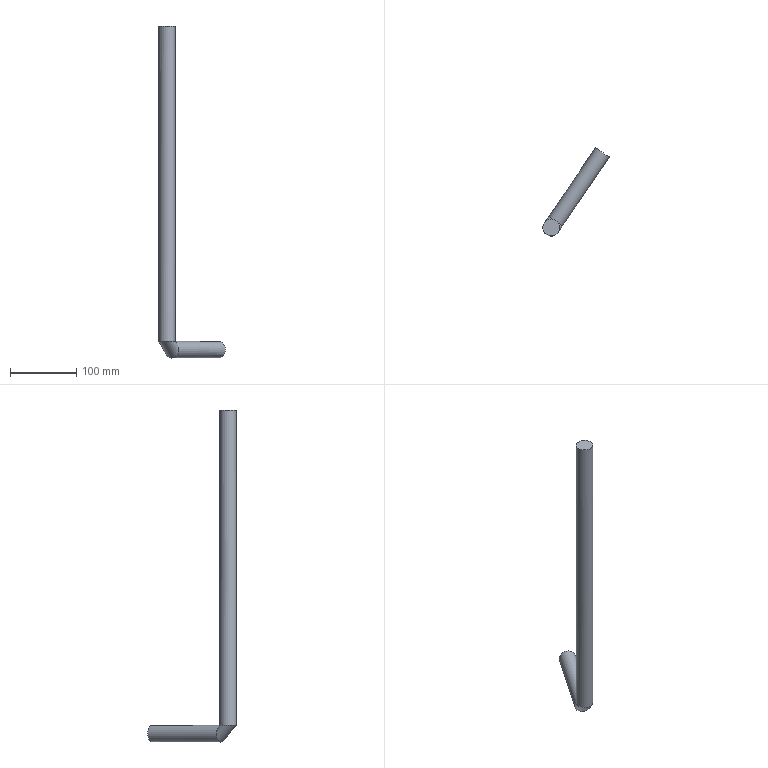Component | NX | PIN | 1 solid | 5 faces | box 100.07 x 133.28 x 500 mm | volume 304163 mm3 | cylinder 2 | plane 2 | torus 1 | commonest cylinder face diameters 25 x2
STEP:
#1=CARTESIAN_POINT('',(0.,0.,0.));
#2=DIRECTION('',(0.,0.,1.));
#3=DIRECTION('',(1.,0.,0.));
#4=AXIS2_PLACEMENT_3D('',#1,#2,#3);
#5=CARTESIAN_POINT('',(-196.929,1175.934,-262.682));
#6=VERTEX_POINT('',#5);
#7=CARTESIAN_POINT('',(-186.587,1168.913,-262.682));
#8=DIRECTION('',(0.5617,0.8274,-0.));
#9=DIRECTION('',(-0.8274,0.5617,0.));
#10=AXIS2_PLACEMENT_3D('',#7,#8,#9);
#11=CIRCLE('',#10,12.5);
#12=CARTESIAN_POINT('',(-256.797,1065.494,-262.682));
#13=DIRECTION('',(0.5617,0.8274,0.));
#14=DIRECTION('',(-0.8274,0.5617,0.));
#15=AXIS2_PLACEMENT_3D('',#12,#13,#14);
#16=CYLINDRICAL_SURFACE('',#15,12.5);
#17=CARTESIAN_POINT('',(0.,125.));
#18=DIRECTION('',(1.,0.));
#19=VECTOR('',#18,1.);
#20=LINE('',#17,#19);
#21=(GEOMETRIC_REPRESENTATION_CONTEXT(2)PARAMETRIC_REPRESENTATION_CONTEXT()REPRESENTATION_CONTEXT('',''));
#22=DEFINITIONAL_REPRESENTATION('',(#20),#21);
#23=PCURVE('',#16,#22);
#24=CARTESIAN_POINT('',(-186.587,1168.913,-262.682));
#25=DIRECTION('',(0.5617,0.8274,-0.));
#26=DIRECTION('',(-0.,-0.,-1.));
#27=AXIS2_PLACEMENT_3D('',#24,#25,#26);
#28=PLANE('',#27);
#29=CARTESIAN_POINT('',(0.,0.));
#30=DIRECTION('',(0.,1.));
#31=AXIS2_PLACEMENT_2D('',#29,#30);
#32=CIRCLE('',#31,12.5);
#33=(GEOMETRIC_REPRESENTATION_CONTEXT(2)PARAMETRIC_REPRESENTATION_CONTEXT()REPRESENTATION_CONTEXT('',''));
#34=DEFINITIONAL_REPRESENTATION('',(#32),#33);
#35=PCURVE('',#28,#34);
#36=SURFACE_CURVE('',#11,(#23,#35),.PCURVE_S1.);
#37=EDGE_CURVE('',#6,#6,#36,.T.);
#38=ORIENTED_EDGE('',*,*,#37,.F.);
#39=CARTESIAN_POINT('',(-267.139,1072.515,-262.682));
#40=VERTEX_POINT('',#39);
#41=CARTESIAN_POINT('',(-267.139,1072.515,-262.682));
#42=CARTESIAN_POINT('',(-196.929,1175.934,-262.682));
#43=B_SPLINE_CURVE_WITH_KNOTS('',1,(#41,#42),.UNSPECIFIED.,.F.,.F.,(2,2),(0.,125.),.PIECEWISE_BEZIER_KNOTS.);
#44=CARTESIAN_POINT('',(0.,0.));
#45=DIRECTION('',(0.,1.));
#46=VECTOR('',#45,1.);
#47=LINE('',#44,#46);
#48=(GEOMETRIC_REPRESENTATION_CONTEXT(2)PARAMETRIC_REPRESENTATION_CONTEXT()REPRESENTATION_CONTEXT('',''));
#49=DEFINITIONAL_REPRESENTATION('',(#47),#48);
#50=PCURVE('',#16,#49);
#51=CARTESIAN_POINT('',(6.283,0.));
#52=DIRECTION('',(0.,1.));
#53=VECTOR('',#52,1.);
#54=LINE('',#51,#53);
#55=(GEOMETRIC_REPRESENTATION_CONTEXT(2)PARAMETRIC_REPRESENTATION_CONTEXT()REPRESENTATION_CONTEXT('',''));
#56=DEFINITIONAL_REPRESENTATION('',(#54),#55);
#57=PCURVE('',#16,#56);
#58=SEAM_CURVE('',#43,(#50,#57),.PCURVE_S1.);
#59=EDGE_CURVE('',#40,#6,#58,.T.);
#60=ORIENTED_EDGE('',*,*,#59,.F.);
#61=CARTESIAN_POINT('',(-256.797,1065.494,-250.182));
#62=VERTEX_POINT('',#61);
#63=CARTESIAN_POINT('',(-256.797,1065.494,-262.682));
#64=DIRECTION('',(0.5617,0.8274,-0.));
#65=DIRECTION('',(-0.8274,0.5617,0.));
#66=AXIS2_PLACEMENT_3D('',#63,#64,#65);
#67=CIRCLE('',#66,12.5);
#68=CARTESIAN_POINT('',(-0.,0.));
#69=DIRECTION('',(1.,0.));
#70=VECTOR('',#69,1.);
#71=LINE('',#68,#70);
#72=(GEOMETRIC_REPRESENTATION_CONTEXT(2)PARAMETRIC_REPRESENTATION_CONTEXT()REPRESENTATION_CONTEXT('',''));
#73=DEFINITIONAL_REPRESENTATION('',(#71),#72);
#74=PCURVE('',#16,#73);
#75=CARTESIAN_POINT('',(-256.797,1065.494,-250.182));
#76=DIRECTION('',(0.8274,-0.5617,0.));
#77=DIRECTION('',(0.5617,0.8274,0.));
#78=AXIS2_PLACEMENT_3D('',#75,#76,#77);
#79=TOROIDAL_SURFACE('',#78,12.5,12.5);
#80=CARTESIAN_POINT('',(4.712,4.712));
#81=DIRECTION('',(0.,-1.));
#82=VECTOR('',#81,1.);
#83=LINE('',#80,#82);
#84=(GEOMETRIC_REPRESENTATION_CONTEXT(2)PARAMETRIC_REPRESENTATION_CONTEXT()REPRESENTATION_CONTEXT('',''));
#85=DEFINITIONAL_REPRESENTATION('',(#83),#84);
#86=PCURVE('',#79,#85);
#87=SURFACE_CURVE('',#67,(#74,#86),.PCURVE_S1.);
#88=EDGE_CURVE('',#40,#62,#87,.T.);
#89=ORIENTED_EDGE('',*,*,#88,.T.);
#90=CARTESIAN_POINT('',(-256.797,1065.494,-262.682));
#91=DIRECTION('',(0.5617,0.8274,-0.));
#92=DIRECTION('',(-0.8274,0.5617,0.));
#93=AXIS2_PLACEMENT_3D('',#90,#91,#92);
#94=CIRCLE('',#93,12.5);
#95=CARTESIAN_POINT('',(-0.,0.));
#96=DIRECTION('',(1.,0.));
#97=VECTOR('',#96,1.);
#98=LINE('',#95,#97);
#99=(GEOMETRIC_REPRESENTATION_CONTEXT(2)PARAMETRIC_REPRESENTATION_CONTEXT()REPRESENTATION_CONTEXT('',''));
#100=DEFINITIONAL_REPRESENTATION('',(#98),#99);
#101=PCURVE('',#16,#100);
#102=CARTESIAN_POINT('',(4.712,10.996));
#103=DIRECTION('',(-0.,-1.));
#104=VECTOR('',#103,1.);
#105=LINE('',#102,#104);
#106=(GEOMETRIC_REPRESENTATION_CONTEXT(2)PARAMETRIC_REPRESENTATION_CONTEXT()REPRESENTATION_CONTEXT('',''));
#107=DEFINITIONAL_REPRESENTATION('',(#105),#106);
#108=PCURVE('',#79,#107);
#109=SURFACE_CURVE('',#94,(#101,#108),.PCURVE_S1.);
#110=EDGE_CURVE('',#62,#40,#109,.T.);
#111=ORIENTED_EDGE('',*,*,#110,.T.);
#112=ORIENTED_EDGE('',*,*,#59,.T.);
#113=EDGE_LOOP('',(#38,#60,#89,#111,#112));
#114=FACE_BOUND('',#113,.T.);
#115=ADVANCED_FACE('',(#114),#16,.T.);
#116=CARTESIAN_POINT('',(-263.818,1055.152,-250.182));
#117=DIRECTION('',(0.,0.,-1.));
#118=DIRECTION('',(-0.8274,0.5617,0.));
#119=AXIS2_PLACEMENT_3D('',#116,#117,#118);
#120=CIRCLE('',#119,12.5);
#121=CARTESIAN_POINT('',(3.142,10.996));
#122=DIRECTION('',(0.,-1.));
#123=VECTOR('',#122,1.);
#124=LINE('',#121,#123);
#125=(GEOMETRIC_REPRESENTATION_CONTEXT(2)PARAMETRIC_REPRESENTATION_CONTEXT()REPRESENTATION_CONTEXT('',''));
#126=DEFINITIONAL_REPRESENTATION('',(#124),#125);
#127=PCURVE('',#79,#126);
#128=CARTESIAN_POINT('',(-263.818,1055.152,-250.182));
#129=DIRECTION('',(0.,0.,1.));
#130=DIRECTION('',(0.5617,0.8274,0.));
#131=AXIS2_PLACEMENT_3D('',#128,#129,#130);
#132=CYLINDRICAL_SURFACE('',#131,12.5);
#133=CARTESIAN_POINT('',(7.854,0.));
#134=DIRECTION('',(-1.,0.));
#135=VECTOR('',#134,1.);
#136=LINE('',#133,#135);
#137=(GEOMETRIC_REPRESENTATION_CONTEXT(2)PARAMETRIC_REPRESENTATION_CONTEXT()REPRESENTATION_CONTEXT('',''));
#138=DEFINITIONAL_REPRESENTATION('',(#136),#137);
#139=PCURVE('',#132,#138);
#140=SURFACE_CURVE('',#120,(#127,#139),.PCURVE_S1.);
#141=EDGE_CURVE('',#62,#62,#140,.T.);
#142=ORIENTED_EDGE('',*,*,#141,.T.);
#143=ORIENTED_EDGE('',*,*,#88,.F.);
#144=ORIENTED_EDGE('',*,*,#110,.F.);
#145=EDGE_LOOP('',(#142,#143,#144));
#146=FACE_BOUND('',#145,.T.);
#147=ADVANCED_FACE('',(#146),#79,.T.);
#148=ORIENTED_EDGE('',*,*,#141,.F.);
#149=CARTESIAN_POINT('',(-256.797,1065.494,224.818));
#150=VERTEX_POINT('',#149);
#151=CARTESIAN_POINT('',(-256.797,1065.494,-250.182));
#152=CARTESIAN_POINT('',(-256.797,1065.494,224.818));
#153=B_SPLINE_CURVE_WITH_KNOTS('',1,(#151,#152),.UNSPECIFIED.,.F.,.F.,(2,2),(0.,475.),.PIECEWISE_BEZIER_KNOTS.);
#154=CARTESIAN_POINT('',(6.283,0.));
#155=DIRECTION('',(0.,1.));
#156=VECTOR('',#155,1.);
#157=LINE('',#154,#156);
#158=(GEOMETRIC_REPRESENTATION_CONTEXT(2)PARAMETRIC_REPRESENTATION_CONTEXT()REPRESENTATION_CONTEXT('',''));
#159=DEFINITIONAL_REPRESENTATION('',(#157),#158);
#160=PCURVE('',#132,#159);
#161=CARTESIAN_POINT('',(0.,0.));
#162=DIRECTION('',(0.,1.));
#163=VECTOR('',#162,1.);
#164=LINE('',#161,#163);
#165=(GEOMETRIC_REPRESENTATION_CONTEXT(2)PARAMETRIC_REPRESENTATION_CONTEXT()REPRESENTATION_CONTEXT('',''));
#166=DEFINITIONAL_REPRESENTATION('',(#164),#165);
#167=PCURVE('',#132,#166);
#168=SEAM_CURVE('',#153,(#160,#167),.PCURVE_S1.);
#169=EDGE_CURVE('',#62,#150,#168,.T.);
#170=ORIENTED_EDGE('',*,*,#169,.T.);
#171=CARTESIAN_POINT('',(-274.16,1062.173,224.818));
#172=VERTEX_POINT('',#171);
#173=CARTESIAN_POINT('',(-263.818,1055.152,224.818));
#174=DIRECTION('',(0.,0.,-1.));
#175=DIRECTION('',(-0.8274,0.5617,0.));
#176=AXIS2_PLACEMENT_3D('',#173,#174,#175);
#177=CIRCLE('',#176,12.5);
#178=CARTESIAN_POINT('',(7.854,475.));
#179=DIRECTION('',(-1.,0.));
#180=VECTOR('',#179,1.);
#181=LINE('',#178,#180);
#182=(GEOMETRIC_REPRESENTATION_CONTEXT(2)PARAMETRIC_REPRESENTATION_CONTEXT()REPRESENTATION_CONTEXT('',''));
#183=DEFINITIONAL_REPRESENTATION('',(#181),#182);
#184=PCURVE('',#132,#183);
#185=CARTESIAN_POINT('',(-263.818,1055.152,224.818));
#186=DIRECTION('',(0.,0.,-1.));
#187=DIRECTION('',(-0.5617,-0.8274,0.));
#188=AXIS2_PLACEMENT_3D('',#185,#186,#187);
#189=PLANE('',#188);
#190=CARTESIAN_POINT('',(0.,0.));
#191=DIRECTION('',(-0.,1.));
#192=AXIS2_PLACEMENT_2D('',#190,#191);
#193=CIRCLE('',#192,12.5);
#194=(GEOMETRIC_REPRESENTATION_CONTEXT(2)PARAMETRIC_REPRESENTATION_CONTEXT()REPRESENTATION_CONTEXT('',''));
#195=DEFINITIONAL_REPRESENTATION('',(#193),#194);
#196=PCURVE('',#189,#195);
#197=SURFACE_CURVE('',#177,(#184,#196),.PCURVE_S1.);
#198=EDGE_CURVE('',#150,#172,#197,.T.);
#199=ORIENTED_EDGE('',*,*,#198,.T.);
#200=CARTESIAN_POINT('',(-263.818,1055.152,224.818));
#201=DIRECTION('',(0.,0.,-1.));
#202=DIRECTION('',(-0.8274,0.5617,0.));
#203=AXIS2_PLACEMENT_3D('',#200,#201,#202);
#204=CIRCLE('',#203,12.5);
#205=CARTESIAN_POINT('',(1.571,475.));
#206=DIRECTION('',(-1.,0.));
#207=VECTOR('',#206,1.);
#208=LINE('',#205,#207);
#209=(GEOMETRIC_REPRESENTATION_CONTEXT(2)PARAMETRIC_REPRESENTATION_CONTEXT()REPRESENTATION_CONTEXT('',''));
#210=DEFINITIONAL_REPRESENTATION('',(#208),#209);
#211=PCURVE('',#132,#210);
#212=CARTESIAN_POINT('',(0.,0.));
#213=DIRECTION('',(-0.,1.));
#214=AXIS2_PLACEMENT_2D('',#212,#213);
#215=CIRCLE('',#214,12.5);
#216=(GEOMETRIC_REPRESENTATION_CONTEXT(2)PARAMETRIC_REPRESENTATION_CONTEXT()REPRESENTATION_CONTEXT('',''));
#217=DEFINITIONAL_REPRESENTATION('',(#215),#216);
#218=PCURVE('',#189,#217);
#219=SURFACE_CURVE('',#204,(#211,#218),.PCURVE_S1.);
#220=EDGE_CURVE('',#172,#150,#219,.T.);
#221=ORIENTED_EDGE('',*,*,#220,.T.);
#222=ORIENTED_EDGE('',*,*,#169,.F.);
#223=EDGE_LOOP('',(#148,#170,#199,#221,#222));
#224=FACE_BOUND('',#223,.T.);
#225=ADVANCED_FACE('',(#224),#132,.T.);
#226=ORIENTED_EDGE('',*,*,#37,.T.);
#227=EDGE_LOOP('',(#226));
#228=FACE_BOUND('',#227,.T.);
#229=ADVANCED_FACE('',(#228),#28,.T.);
#230=ORIENTED_EDGE('',*,*,#220,.F.);
#231=ORIENTED_EDGE('',*,*,#198,.F.);
#232=EDGE_LOOP('',(#230,#231));
#233=FACE_BOUND('',#232,.T.);
#234=ADVANCED_FACE('',(#233),#189,.F.);
#235=CLOSED_SHELL('',(#115,#147,#225,#229,#234));
#236=MANIFOLD_SOLID_BREP('',#235);
#237=(LENGTH_UNIT()NAMED_UNIT(*)SI_UNIT(.MILLI.,.METRE.));
#238=UNCERTAINTY_MEASURE_WITH_UNIT(LENGTH_MEASURE(0.000005),#237,'','');
#239=(NAMED_UNIT(*)PLANE_ANGLE_UNIT()SI_UNIT($,.RADIAN.));
#240=(NAMED_UNIT(*)SI_UNIT($,.STERADIAN.)SOLID_ANGLE_UNIT());
#241=(GEOMETRIC_REPRESENTATION_CONTEXT(3)GLOBAL_UNCERTAINTY_ASSIGNED_CONTEXT((#238))GLOBAL_UNIT_ASSIGNED_CONTEXT((#237,#239,#240))REPRESENTATION_CONTEXT('',''));
#242=ADVANCED_BREP_SHAPE_REPRESENTATION('',(#4,#236),#241);